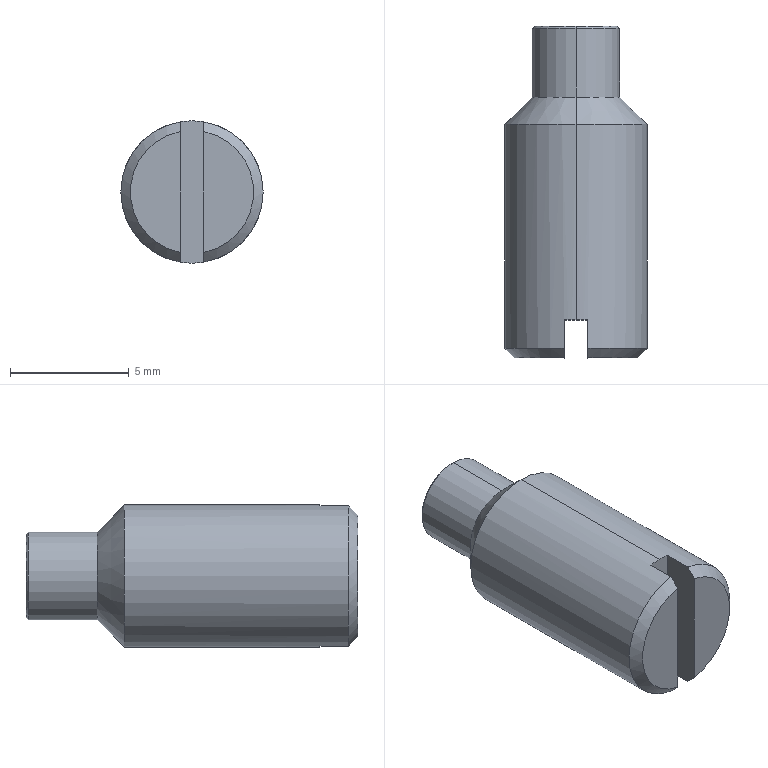Component | NX | GB_T_75_1985_SLOTTEDSETSCREW_M6X14 | 1 solid | 16 faces | box 6 x 14 x 6 mm | volume 321 mm3 | cone 6 | plane 6 | cylinder 4 | commonest cylinder face diameters 3.7 x2 6 x2
STEP:
#1=CARTESIAN_POINT('',(0.,0.,0.));
#2=DIRECTION('',(0.,0.,1.));
#3=DIRECTION('',(1.,0.,0.));
#4=AXIS2_PLACEMENT_3D('',#1,#2,#3);
#5=CARTESIAN_POINT('',(4.835,-12.785,234.25));
#6=VERTEX_POINT('',#5);
#7=CARTESIAN_POINT('',(4.835,-12.785,237.75));
#8=VERTEX_POINT('',#7);
#9=CARTESIAN_POINT('',(4.835,-12.785,236.));
#10=DIRECTION('',(0.,1.,0.));
#11=DIRECTION('',(0.,0.,1.));
#12=AXIS2_PLACEMENT_3D('',#9,#10,#11);
#13=CIRCLE('',#12,1.75);
#14=CARTESIAN_POINT('',(4.835,-12.885,236.));
#15=DIRECTION('',(0.,-1.,0.));
#16=DIRECTION('',(0.,0.,-1.));
#17=AXIS2_PLACEMENT_3D('',#14,#15,#16);
#18=CONICAL_SURFACE('',#17,1.85,0.7854);
#19=CARTESIAN_POINT('',(9.425,-0.1));
#20=DIRECTION('',(-1.,0.));
#21=VECTOR('',#20,1.);
#22=LINE('',#19,#21);
#23=(GEOMETRIC_REPRESENTATION_CONTEXT(2)PARAMETRIC_REPRESENTATION_CONTEXT()REPRESENTATION_CONTEXT('',''));
#24=DEFINITIONAL_REPRESENTATION('',(#22),#23);
#25=PCURVE('',#18,#24);
#26=CARTESIAN_POINT('',(2.985,-12.785,236.));
#27=DIRECTION('',(0.,-1.,0.));
#28=DIRECTION('',(0.,0.,-1.));
#29=AXIS2_PLACEMENT_3D('',#26,#27,#28);
#30=PLANE('',#29);
#31=CARTESIAN_POINT('',(-1.75,1.85));
#32=CARTESIAN_POINT('',(-1.75,4.881));
#33=CARTESIAN_POINT('',(0.875,3.366));
#34=CARTESIAN_POINT('',(3.5,1.85));
#35=CARTESIAN_POINT('',(0.875,0.3345));
#36=CARTESIAN_POINT('',(-1.75,-1.181));
#37=CARTESIAN_POINT('',(-1.75,1.85));
#38=(BOUNDED_CURVE()B_SPLINE_CURVE(2,(#31,#32,#33,#34,#35,#36,#37),.UNSPECIFIED.,.T.,.F.)B_SPLINE_CURVE_WITH_KNOTS((1,2,2,2,2,1),(-2.094,0.,2.094,4.189,6.283,8.378),.UNSPECIFIED.)CURVE()GEOMETRIC_REPRESENTATION_ITEM()RATIONAL_B_SPLINE_CURVE((1.,0.5,1.,0.5,1.,0.5,1.))REPRESENTATION_ITEM(''));
#39=(GEOMETRIC_REPRESENTATION_CONTEXT(2)PARAMETRIC_REPRESENTATION_CONTEXT()REPRESENTATION_CONTEXT('',''));
#40=DEFINITIONAL_REPRESENTATION('',(#38),#39);
#41=PCURVE('',#30,#40);
#42=SURFACE_CURVE('',#13,(#25,#41),.PCURVE_S1.);
#43=EDGE_CURVE('',#6,#8,#42,.T.);
#44=ORIENTED_EDGE('',*,*,#43,.F.);
#45=CARTESIAN_POINT('',(4.835,-12.885,234.15));
#46=VERTEX_POINT('',#45);
#47=CARTESIAN_POINT('',(4.835,-12.885,234.15));
#48=DIRECTION('',(-0.,-0.7071,-0.7071));
#49=VECTOR('',#48,1.);
#50=LINE('',#47,#49);
#51=CARTESIAN_POINT('',(6.283,-0.));
#52=DIRECTION('',(0.,1.));
#53=VECTOR('',#52,1.);
#54=LINE('',#51,#53);
#55=(GEOMETRIC_REPRESENTATION_CONTEXT(2)PARAMETRIC_REPRESENTATION_CONTEXT()REPRESENTATION_CONTEXT('',''));
#56=DEFINITIONAL_REPRESENTATION('',(#54),#55);
#57=PCURVE('',#18,#56);
#58=CARTESIAN_POINT('',(4.835,-12.885,236.));
#59=DIRECTION('',(0.,-1.,0.));
#60=DIRECTION('',(0.,0.,-1.));
#61=AXIS2_PLACEMENT_3D('',#58,#59,#60);
#62=CONICAL_SURFACE('',#61,1.85,0.7854);
#63=CARTESIAN_POINT('',(0.,-0.));
#64=DIRECTION('',(0.,1.));
#65=VECTOR('',#64,1.);
#66=LINE('',#63,#65);
#67=(GEOMETRIC_REPRESENTATION_CONTEXT(2)PARAMETRIC_REPRESENTATION_CONTEXT()REPRESENTATION_CONTEXT('',''));
#68=DEFINITIONAL_REPRESENTATION('',(#66),#67);
#69=PCURVE('',#62,#68);
#70=SURFACE_CURVE('',#50,(#57,#69),.PCURVE_S1.);
#71=EDGE_CURVE('',#6,#46,#70,.T.);
#72=ORIENTED_EDGE('',*,*,#71,.T.);
#73=CARTESIAN_POINT('',(4.835,-12.885,237.85));
#74=VERTEX_POINT('',#73);
#75=CARTESIAN_POINT('',(4.835,-12.885,236.));
#76=DIRECTION('',(0.,-1.,0.));
#77=DIRECTION('',(0.,0.,1.));
#78=AXIS2_PLACEMENT_3D('',#75,#76,#77);
#79=CIRCLE('',#78,1.85);
#80=CARTESIAN_POINT('',(3.142,-0.));
#81=DIRECTION('',(1.,0.));
#82=VECTOR('',#81,1.);
#83=LINE('',#80,#82);
#84=(GEOMETRIC_REPRESENTATION_CONTEXT(2)PARAMETRIC_REPRESENTATION_CONTEXT()REPRESENTATION_CONTEXT('',''));
#85=DEFINITIONAL_REPRESENTATION('',(#83),#84);
#86=PCURVE('',#18,#85);
#87=CARTESIAN_POINT('',(4.835,-28.21,236.));
#88=DIRECTION('',(0.,-1.,0.));
#89=DIRECTION('',(0.,0.,-1.));
#90=AXIS2_PLACEMENT_3D('',#87,#88,#89);
#91=CYLINDRICAL_SURFACE('',#90,1.85);
#92=CARTESIAN_POINT('',(3.142,-15.325));
#93=DIRECTION('',(1.,0.));
#94=VECTOR('',#93,1.);
#95=LINE('',#92,#94);
#96=(GEOMETRIC_REPRESENTATION_CONTEXT(2)PARAMETRIC_REPRESENTATION_CONTEXT()REPRESENTATION_CONTEXT('',''));
#97=DEFINITIONAL_REPRESENTATION('',(#95),#96);
#98=PCURVE('',#91,#97);
#99=SURFACE_CURVE('',#79,(#86,#98),.PCURVE_S1.);
#100=EDGE_CURVE('',#74,#46,#99,.T.);
#101=ORIENTED_EDGE('',*,*,#100,.F.);
#102=CARTESIAN_POINT('',(4.835,-12.885,237.85));
#103=DIRECTION('',(0.,-0.7071,0.7071));
#104=VECTOR('',#103,1.);
#105=LINE('',#102,#104);
#106=CARTESIAN_POINT('',(3.142,-0.));
#107=DIRECTION('',(0.,1.));
#108=VECTOR('',#107,1.);
#109=LINE('',#106,#108);
#110=(GEOMETRIC_REPRESENTATION_CONTEXT(2)PARAMETRIC_REPRESENTATION_CONTEXT()REPRESENTATION_CONTEXT('',''));
#111=DEFINITIONAL_REPRESENTATION('',(#109),#110);
#112=PCURVE('',#18,#111);
#113=CARTESIAN_POINT('',(3.142,-0.));
#114=DIRECTION('',(0.,1.));
#115=VECTOR('',#114,1.);
#116=LINE('',#113,#115);
#117=(GEOMETRIC_REPRESENTATION_CONTEXT(2)PARAMETRIC_REPRESENTATION_CONTEXT()REPRESENTATION_CONTEXT('',''));
#118=DEFINITIONAL_REPRESENTATION('',(#116),#117);
#119=PCURVE('',#62,#118);
#120=SURFACE_CURVE('',#105,(#112,#119),.PCURVE_S1.);
#121=EDGE_CURVE('',#8,#74,#120,.T.);
#122=ORIENTED_EDGE('',*,*,#121,.F.);
#123=EDGE_LOOP('',(#44,#72,#101,#122));
#124=FACE_BOUND('',#123,.T.);
#125=ADVANCED_FACE('',(#124),#18,.T.);
#126=ORIENTED_EDGE('',*,*,#100,.T.);
#127=CARTESIAN_POINT('',(4.835,-15.785,234.15));
#128=VERTEX_POINT('',#127);
#129=CARTESIAN_POINT('',(4.835,-28.21,234.15));
#130=DIRECTION('',(0.,-1.,0.));
#131=VECTOR('',#130,1.);
#132=LINE('',#129,#131);
#133=CARTESIAN_POINT('',(6.283,0.));
#134=DIRECTION('',(0.,1.));
#135=VECTOR('',#134,1.);
#136=LINE('',#133,#135);
#137=(GEOMETRIC_REPRESENTATION_CONTEXT(2)PARAMETRIC_REPRESENTATION_CONTEXT()REPRESENTATION_CONTEXT('',''));
#138=DEFINITIONAL_REPRESENTATION('',(#136),#137);
#139=PCURVE('',#91,#138);
#140=CARTESIAN_POINT('',(4.835,-28.21,236.));
#141=DIRECTION('',(0.,-1.,0.));
#142=DIRECTION('',(0.,0.,-1.));
#143=AXIS2_PLACEMENT_3D('',#140,#141,#142);
#144=CYLINDRICAL_SURFACE('',#143,1.85);
#145=CARTESIAN_POINT('',(0.,0.));
#146=DIRECTION('',(0.,1.));
#147=VECTOR('',#146,1.);
#148=LINE('',#145,#147);
#149=(GEOMETRIC_REPRESENTATION_CONTEXT(2)PARAMETRIC_REPRESENTATION_CONTEXT()REPRESENTATION_CONTEXT('',''));
#150=DEFINITIONAL_REPRESENTATION('',(#148),#149);
#151=PCURVE('',#144,#150);
#152=SURFACE_CURVE('',#132,(#139,#151),.PCURVE_S1.);
#153=EDGE_CURVE('',#46,#128,#152,.T.);
#154=ORIENTED_EDGE('',*,*,#153,.T.);
#155=CARTESIAN_POINT('',(4.835,-15.785,237.85));
#156=VERTEX_POINT('',#155);
#157=CARTESIAN_POINT('',(4.835,-15.785,236.));
#158=DIRECTION('',(0.,-1.,0.));
#159=DIRECTION('',(0.,0.,1.));
#160=AXIS2_PLACEMENT_3D('',#157,#158,#159);
#161=CIRCLE('',#160,1.85);
#162=CARTESIAN_POINT('',(3.142,-12.425));
#163=DIRECTION('',(1.,0.));
#164=VECTOR('',#163,1.);
#165=LINE('',#162,#164);
#166=(GEOMETRIC_REPRESENTATION_CONTEXT(2)PARAMETRIC_REPRESENTATION_CONTEXT()REPRESENTATION_CONTEXT('',''));
#167=DEFINITIONAL_REPRESENTATION('',(#165),#166);
#168=PCURVE('',#91,#167);
#169=CARTESIAN_POINT('',(4.835,-15.785,236.));
#170=DIRECTION('',(0.,-1.,0.));
#171=DIRECTION('',(0.,0.,-1.));
#172=AXIS2_PLACEMENT_3D('',#169,#170,#171);
#173=CONICAL_SURFACE('',#172,1.85,0.7854);
#174=CARTESIAN_POINT('',(3.142,-0.));
#175=DIRECTION('',(1.,0.));
#176=VECTOR('',#175,1.);
#177=LINE('',#174,#176);
#178=(GEOMETRIC_REPRESENTATION_CONTEXT(2)PARAMETRIC_REPRESENTATION_CONTEXT()REPRESENTATION_CONTEXT('',''));
#179=DEFINITIONAL_REPRESENTATION('',(#177),#178);
#180=PCURVE('',#173,#179);
#181=SURFACE_CURVE('',#161,(#168,#180),.PCURVE_S1.);
#182=EDGE_CURVE('',#156,#128,#181,.T.);
#183=ORIENTED_EDGE('',*,*,#182,.F.);
#184=CARTESIAN_POINT('',(4.835,-28.21,237.85));
#185=DIRECTION('',(0.,-1.,0.));
#186=VECTOR('',#185,1.);
#187=LINE('',#184,#186);
#188=CARTESIAN_POINT('',(3.142,0.));
#189=DIRECTION('',(0.,1.));
#190=VECTOR('',#189,1.);
#191=LINE('',#188,#190);
#192=(GEOMETRIC_REPRESENTATION_CONTEXT(2)PARAMETRIC_REPRESENTATION_CONTEXT()REPRESENTATION_CONTEXT('',''));
#193=DEFINITIONAL_REPRESENTATION('',(#191),#192);
#194=PCURVE('',#91,#193);
#195=CARTESIAN_POINT('',(3.142,0.));
#196=DIRECTION('',(0.,1.));
#197=VECTOR('',#196,1.);
#198=LINE('',#195,#197);
#199=(GEOMETRIC_REPRESENTATION_CONTEXT(2)PARAMETRIC_REPRESENTATION_CONTEXT()REPRESENTATION_CONTEXT('',''));
#200=DEFINITIONAL_REPRESENTATION('',(#198),#199);
#201=PCURVE('',#144,#200);
#202=SURFACE_CURVE('',#187,(#194,#201),.PCURVE_S1.);
#203=EDGE_CURVE('',#74,#156,#202,.T.);
#204=ORIENTED_EDGE('',*,*,#203,.F.);
#205=EDGE_LOOP('',(#126,#154,#183,#204));
#206=FACE_BOUND('',#205,.T.);
#207=ADVANCED_FACE('',(#206),#91,.T.);
#208=ORIENTED_EDGE('',*,*,#182,.T.);
#209=CARTESIAN_POINT('',(4.835,-16.935,233.));
#210=VERTEX_POINT('',#209);
#211=CARTESIAN_POINT('',(4.835,-15.785,234.15));
#212=DIRECTION('',(-0.,-0.7071,-0.7071));
#213=VECTOR('',#212,1.);
#214=LINE('',#211,#213);
#215=CARTESIAN_POINT('',(6.283,-0.));
#216=DIRECTION('',(0.,1.));
#217=VECTOR('',#216,1.);
#218=LINE('',#215,#217);
#219=(GEOMETRIC_REPRESENTATION_CONTEXT(2)PARAMETRIC_REPRESENTATION_CONTEXT()REPRESENTATION_CONTEXT('',''));
#220=DEFINITIONAL_REPRESENTATION('',(#218),#219);
#221=PCURVE('',#173,#220);
#222=CARTESIAN_POINT('',(4.835,-15.785,236.));
#223=DIRECTION('',(0.,-1.,0.));
#224=DIRECTION('',(0.,0.,-1.));
#225=AXIS2_PLACEMENT_3D('',#222,#223,#224);
#226=CONICAL_SURFACE('',#225,1.85,0.7854);
#227=CARTESIAN_POINT('',(0.,-0.));
#228=DIRECTION('',(0.,1.));
#229=VECTOR('',#228,1.);
#230=LINE('',#227,#229);
#231=(GEOMETRIC_REPRESENTATION_CONTEXT(2)PARAMETRIC_REPRESENTATION_CONTEXT()REPRESENTATION_CONTEXT('',''));
#232=DEFINITIONAL_REPRESENTATION('',(#230),#231);
#233=PCURVE('',#226,#232);
#234=SURFACE_CURVE('',#214,(#221,#233),.PCURVE_S1.);
#235=EDGE_CURVE('',#128,#210,#234,.T.);
#236=ORIENTED_EDGE('',*,*,#235,.T.);
#237=CARTESIAN_POINT('',(4.835,-16.935,239.));
#238=VERTEX_POINT('',#237);
#239=CARTESIAN_POINT('',(4.835,-16.935,236.));
#240=DIRECTION('',(0.,-1.,0.));
#241=DIRECTION('',(0.,0.,1.));
#242=AXIS2_PLACEMENT_3D('',#239,#240,#241);
#243=CIRCLE('',#242,3.);
#244=CARTESIAN_POINT('',(3.142,1.15));
#245=DIRECTION('',(1.,0.));
#246=VECTOR('',#245,1.);
#247=LINE('',#244,#246);
#248=(GEOMETRIC_REPRESENTATION_CONTEXT(2)PARAMETRIC_REPRESENTATION_CONTEXT()REPRESENTATION_CONTEXT('',''));
#249=DEFINITIONAL_REPRESENTATION('',(#247),#248);
#250=PCURVE('',#173,#249);
#251=CARTESIAN_POINT('',(4.835,-28.21,236.));
#252=DIRECTION('',(0.,-1.,0.));
#253=DIRECTION('',(0.,0.,-1.));
#254=AXIS2_PLACEMENT_3D('',#251,#252,#253);
#255=CYLINDRICAL_SURFACE('',#254,3.);
#256=CARTESIAN_POINT('',(3.142,-11.275));
#257=DIRECTION('',(1.,0.));
#258=VECTOR('',#257,1.);
#259=LINE('',#256,#258);
#260=(GEOMETRIC_REPRESENTATION_CONTEXT(2)PARAMETRIC_REPRESENTATION_CONTEXT()REPRESENTATION_CONTEXT('',''));
#261=DEFINITIONAL_REPRESENTATION('',(#259),#260);
#262=PCURVE('',#255,#261);
#263=SURFACE_CURVE('',#243,(#250,#262),.PCURVE_S1.);
#264=EDGE_CURVE('',#238,#210,#263,.T.);
#265=ORIENTED_EDGE('',*,*,#264,.F.);
#266=CARTESIAN_POINT('',(4.835,-15.785,237.85));
#267=DIRECTION('',(0.,-0.7071,0.7071));
#268=VECTOR('',#267,1.);
#269=LINE('',#266,#268);
#270=CARTESIAN_POINT('',(3.142,-0.));
#271=DIRECTION('',(0.,1.));
#272=VECTOR('',#271,1.);
#273=LINE('',#270,#272);
#274=(GEOMETRIC_REPRESENTATION_CONTEXT(2)PARAMETRIC_REPRESENTATION_CONTEXT()REPRESENTATION_CONTEXT('',''));
#275=DEFINITIONAL_REPRESENTATION('',(#273),#274);
#276=PCURVE('',#173,#275);
#277=CARTESIAN_POINT('',(3.142,-0.));
#278=DIRECTION('',(0.,1.));
#279=VECTOR('',#278,1.);
#280=LINE('',#277,#279);
#281=(GEOMETRIC_REPRESENTATION_CONTEXT(2)PARAMETRIC_REPRESENTATION_CONTEXT()REPRESENTATION_CONTEXT('',''));
#282=DEFINITIONAL_REPRESENTATION('',(#280),#281);
#283=PCURVE('',#226,#282);
#284=SURFACE_CURVE('',#269,(#276,#283),.PCURVE_S1.);
#285=EDGE_CURVE('',#156,#238,#284,.T.);
#286=ORIENTED_EDGE('',*,*,#285,.F.);
#287=EDGE_LOOP('',(#208,#236,#265,#286));
#288=FACE_BOUND('',#287,.T.);
#289=ADVANCED_FACE('',(#288),#173,.T.);
#290=ORIENTED_EDGE('',*,*,#264,.T.);
#291=CARTESIAN_POINT('',(4.835,-25.185,233.));
#292=VERTEX_POINT('',#291);
#293=CARTESIAN_POINT('',(4.835,-28.21,233.));
#294=DIRECTION('',(0.,-1.,0.));
#295=VECTOR('',#294,1.);
#296=LINE('',#293,#295);
#297=CARTESIAN_POINT('',(6.283,0.));
#298=DIRECTION('',(0.,1.));
#299=VECTOR('',#298,1.);
#300=LINE('',#297,#299);
#301=(GEOMETRIC_REPRESENTATION_CONTEXT(2)PARAMETRIC_REPRESENTATION_CONTEXT()REPRESENTATION_CONTEXT('',''));
#302=DEFINITIONAL_REPRESENTATION('',(#300),#301);
#303=PCURVE('',#255,#302);
#304=CARTESIAN_POINT('',(4.835,-28.21,236.));
#305=DIRECTION('',(0.,-1.,0.));
#306=DIRECTION('',(0.,0.,-1.));
#307=AXIS2_PLACEMENT_3D('',#304,#305,#306);
#308=CYLINDRICAL_SURFACE('',#307,3.);
#309=CARTESIAN_POINT('',(0.,0.));
#310=DIRECTION('',(0.,1.));
#311=VECTOR('',#310,1.);
#312=LINE('',#309,#311);
#313=(GEOMETRIC_REPRESENTATION_CONTEXT(2)PARAMETRIC_REPRESENTATION_CONTEXT()REPRESENTATION_CONTEXT('',''));
#314=DEFINITIONAL_REPRESENTATION('',(#312),#313);
#315=PCURVE('',#308,#314);
#316=SURFACE_CURVE('',#296,(#303,#315),.PCURVE_S1.);
#317=EDGE_CURVE('',#210,#292,#316,.T.);
#318=ORIENTED_EDGE('',*,*,#317,.T.);
#319=CARTESIAN_POINT('',(4.335,-25.185,233.042));
#320=VERTEX_POINT('',#319);
#321=CARTESIAN_POINT('',(4.835,-25.185,236.));
#322=DIRECTION('',(0.,1.,0.));
#323=DIRECTION('',(0.,0.,-1.));
#324=AXIS2_PLACEMENT_3D('',#321,#322,#323);
#325=CIRCLE('',#324,3.);
#326=CARTESIAN_POINT('',(6.283,-3.025));
#327=DIRECTION('',(-1.,0.));
#328=VECTOR('',#327,1.);
#329=LINE('',#326,#328);
#330=(GEOMETRIC_REPRESENTATION_CONTEXT(2)PARAMETRIC_REPRESENTATION_CONTEXT()REPRESENTATION_CONTEXT('',''));
#331=DEFINITIONAL_REPRESENTATION('',(#329),#330);
#332=PCURVE('',#255,#331);
#333=CARTESIAN_POINT('',(4.335,-25.185,186.));
#334=DIRECTION('',(0.,1.,0.));
#335=DIRECTION('',(0.,0.,1.));
#336=AXIS2_PLACEMENT_3D('',#333,#334,#335);
#337=PLANE('',#336);
#338=CARTESIAN_POINT('',(50.,0.5));
#339=DIRECTION('',(-1.,0.));
#340=AXIS2_PLACEMENT_2D('',#338,#339);
#341=CIRCLE('',#340,3.);
#342=(GEOMETRIC_REPRESENTATION_CONTEXT(2)PARAMETRIC_REPRESENTATION_CONTEXT()REPRESENTATION_CONTEXT('',''));
#343=DEFINITIONAL_REPRESENTATION('',(#341),#342);
#344=PCURVE('',#337,#343);
#345=SURFACE_CURVE('',#325,(#332,#344),.PCURVE_S1.);
#346=EDGE_CURVE('',#292,#320,#345,.T.);
#347=ORIENTED_EDGE('',*,*,#346,.T.);
#348=CARTESIAN_POINT('',(4.335,-26.383,233.042));
#349=VERTEX_POINT('',#348);
#350=CARTESIAN_POINT('',(4.335,-28.21,233.042));
#351=DIRECTION('',(0.,-1.,0.));
#352=VECTOR('',#351,1.);
#353=LINE('',#350,#352);
#354=CARTESIAN_POINT('',(6.116,0.));
#355=DIRECTION('',(0.,1.));
#356=VECTOR('',#355,1.);
#357=LINE('',#354,#356);
#358=(GEOMETRIC_REPRESENTATION_CONTEXT(2)PARAMETRIC_REPRESENTATION_CONTEXT()REPRESENTATION_CONTEXT('',''));
#359=DEFINITIONAL_REPRESENTATION('',(#357),#358);
#360=PCURVE('',#255,#359);
#361=CARTESIAN_POINT('',(4.335,-26.785,186.));
#362=DIRECTION('',(-1.,0.,0.));
#363=DIRECTION('',(0.,0.,-1.));
#364=AXIS2_PLACEMENT_3D('',#361,#362,#363);
#365=PLANE('',#364);
#366=CARTESIAN_POINT('',(-47.042,1.425));
#367=DIRECTION('',(0.,1.));
#368=VECTOR('',#367,1.);
#369=LINE('',#366,#368);
#370=(GEOMETRIC_REPRESENTATION_CONTEXT(2)PARAMETRIC_REPRESENTATION_CONTEXT()REPRESENTATION_CONTEXT('',''));
#371=DEFINITIONAL_REPRESENTATION('',(#369),#370);
#372=PCURVE('',#365,#371);
#373=SURFACE_CURVE('',#353,(#360,#372),.PCURVE_S1.);
#374=EDGE_CURVE('',#320,#349,#373,.T.);
#375=ORIENTED_EDGE('',*,*,#374,.T.);
#376=CARTESIAN_POINT('',(4.335,-26.383,238.958));
#377=VERTEX_POINT('',#376);
#378=CARTESIAN_POINT('',(4.835,-26.383,236.));
#379=DIRECTION('',(0.,-1.,0.));
#380=DIRECTION('',(0.,0.,1.));
#381=AXIS2_PLACEMENT_3D('',#378,#379,#380);
#382=CIRCLE('',#381,3.);
#383=CARTESIAN_POINT('',(3.142,-1.827));
#384=DIRECTION('',(1.,0.));
#385=VECTOR('',#384,1.);
#386=LINE('',#383,#385);
#387=(GEOMETRIC_REPRESENTATION_CONTEXT(2)PARAMETRIC_REPRESENTATION_CONTEXT()REPRESENTATION_CONTEXT('',''));
#388=DEFINITIONAL_REPRESENTATION('',(#386),#387);
#389=PCURVE('',#255,#388);
#390=CARTESIAN_POINT('',(4.835,-26.383,236.));
#391=DIRECTION('',(0.,1.,0.));
#392=DIRECTION('',(0.,0.,1.));
#393=AXIS2_PLACEMENT_3D('',#390,#391,#392);
#394=CONICAL_SURFACE('',#393,3.,0.7854);
#395=CARTESIAN_POINT('',(6.283,0.));
#396=DIRECTION('',(-1.,0.));
#397=VECTOR('',#396,1.);
#398=LINE('',#395,#397);
#399=(GEOMETRIC_REPRESENTATION_CONTEXT(2)PARAMETRIC_REPRESENTATION_CONTEXT()REPRESENTATION_CONTEXT('',''));
#400=DEFINITIONAL_REPRESENTATION('',(#398),#399);
#401=PCURVE('',#394,#400);
#402=SURFACE_CURVE('',#382,(#389,#401),.PCURVE_S1.);
#403=EDGE_CURVE('',#377,#349,#402,.T.);
#404=ORIENTED_EDGE('',*,*,#403,.F.);
#405=CARTESIAN_POINT('',(4.335,-25.185,238.958));
#406=VERTEX_POINT('',#405);
#407=CARTESIAN_POINT('',(4.335,-28.21,238.958));
#408=DIRECTION('',(0.,1.,0.));
#409=VECTOR('',#408,1.);
#410=LINE('',#407,#409);
#411=CARTESIAN_POINT('',(3.309,0.));
#412=DIRECTION('',(0.,-1.));
#413=VECTOR('',#412,1.);
#414=LINE('',#411,#413);
#415=(GEOMETRIC_REPRESENTATION_CONTEXT(2)PARAMETRIC_REPRESENTATION_CONTEXT()REPRESENTATION_CONTEXT('',''));
#416=DEFINITIONAL_REPRESENTATION('',(#414),#415);
#417=PCURVE('',#255,#416);
#418=CARTESIAN_POINT('',(-52.958,1.425));
#419=DIRECTION('',(0.,-1.));
#420=VECTOR('',#419,1.);
#421=LINE('',#418,#420);
#422=(GEOMETRIC_REPRESENTATION_CONTEXT(2)PARAMETRIC_REPRESENTATION_CONTEXT()REPRESENTATION_CONTEXT('',''));
#423=DEFINITIONAL_REPRESENTATION('',(#421),#422);
#424=PCURVE('',#365,#423);
#425=SURFACE_CURVE('',#410,(#417,#424),.PCURVE_S1.);
#426=EDGE_CURVE('',#377,#406,#425,.T.);
#427=ORIENTED_EDGE('',*,*,#426,.T.);
#428=CARTESIAN_POINT('',(4.835,-25.185,239.));
#429=VERTEX_POINT('',#428);
#430=CARTESIAN_POINT('',(4.835,-25.185,236.));
#431=DIRECTION('',(0.,1.,0.));
#432=DIRECTION('',(0.,0.,-1.));
#433=AXIS2_PLACEMENT_3D('',#430,#431,#432);
#434=CIRCLE('',#433,3.);
#435=CARTESIAN_POINT('',(6.283,-3.025));
#436=DIRECTION('',(-1.,0.));
#437=VECTOR('',#436,1.);
#438=LINE('',#435,#437);
#439=(GEOMETRIC_REPRESENTATION_CONTEXT(2)PARAMETRIC_REPRESENTATION_CONTEXT()REPRESENTATION_CONTEXT('',''));
#440=DEFINITIONAL_REPRESENTATION('',(#438),#439);
#441=PCURVE('',#255,#440);
#442=CARTESIAN_POINT('',(50.,0.5));
#443=DIRECTION('',(-1.,0.));
#444=AXIS2_PLACEMENT_2D('',#442,#443);
#445=CIRCLE('',#444,3.);
#446=(GEOMETRIC_REPRESENTATION_CONTEXT(2)PARAMETRIC_REPRESENTATION_CONTEXT()REPRESENTATION_CONTEXT('',''));
#447=DEFINITIONAL_REPRESENTATION('',(#445),#446);
#448=PCURVE('',#337,#447);
#449=SURFACE_CURVE('',#434,(#441,#448),.PCURVE_S1.);
#450=EDGE_CURVE('',#406,#429,#449,.T.);
#451=ORIENTED_EDGE('',*,*,#450,.T.);
#452=CARTESIAN_POINT('',(4.835,-28.21,239.));
#453=DIRECTION('',(0.,-1.,0.));
#454=VECTOR('',#453,1.);
#455=LINE('',#452,#454);
#456=CARTESIAN_POINT('',(3.142,0.));
#457=DIRECTION('',(0.,1.));
#458=VECTOR('',#457,1.);
#459=LINE('',#456,#458);
#460=(GEOMETRIC_REPRESENTATION_CONTEXT(2)PARAMETRIC_REPRESENTATION_CONTEXT()REPRESENTATION_CONTEXT('',''));
#461=DEFINITIONAL_REPRESENTATION('',(#459),#460);
#462=PCURVE('',#255,#461);
#463=CARTESIAN_POINT('',(3.142,0.));
#464=DIRECTION('',(0.,1.));
#465=VECTOR('',#464,1.);
#466=LINE('',#463,#465);
#467=(GEOMETRIC_REPRESENTATION_CONTEXT(2)PARAMETRIC_REPRESENTATION_CONTEXT()REPRESENTATION_CONTEXT('',''));
#468=DEFINITIONAL_REPRESENTATION('',(#466),#467);
#469=PCURVE('',#308,#468);
#470=SURFACE_CURVE('',#455,(#462,#469),.PCURVE_S1.);
#471=EDGE_CURVE('',#238,#429,#470,.T.);
#472=ORIENTED_EDGE('',*,*,#471,.F.);
#473=EDGE_LOOP('',(#290,#318,#347,#375,#404,#427,#451,#472));
#474=FACE_BOUND('',#473,.T.);
#475=ADVANCED_FACE('',(#474),#255,.T.);
#476=CARTESIAN_POINT('',(4.335,-26.785,238.549));
#477=VERTEX_POINT('',#476);
#478=CARTESIAN_POINT('',(4.335,-26.785,233.451));
#479=VERTEX_POINT('',#478);
#480=CARTESIAN_POINT('',(4.835,-26.785,236.));
#481=DIRECTION('',(0.,-1.,0.));
#482=DIRECTION('',(0.,0.,1.));
#483=AXIS2_PLACEMENT_3D('',#480,#481,#482);
#484=CIRCLE('',#483,2.598);
#485=CARTESIAN_POINT('',(4.835,-26.785,236.));
#486=DIRECTION('',(0.,1.,0.));
#487=DIRECTION('',(0.,0.,1.));
#488=AXIS2_PLACEMENT_3D('',#485,#486,#487);
#489=PLANE('',#488);
#490=CARTESIAN_POINT('',(2.598,0.));
#491=CARTESIAN_POINT('',(2.598,-4.5));
#492=CARTESIAN_POINT('',(-1.299,-2.25));
#493=CARTESIAN_POINT('',(-5.196,-0.));
#494=CARTESIAN_POINT('',(-1.299,2.25));
#495=CARTESIAN_POINT('',(2.598,4.5));
#496=CARTESIAN_POINT('',(2.598,0.));
#497=(BOUNDED_CURVE()B_SPLINE_CURVE(2,(#490,#491,#492,#493,#494,#495,#496),.UNSPECIFIED.,.T.,.F.)B_SPLINE_CURVE_WITH_KNOTS((1,2,2,2,2,1),(-2.094,0.,2.094,4.189,6.283,8.378),.UNSPECIFIED.)CURVE()GEOMETRIC_REPRESENTATION_ITEM()RATIONAL_B_SPLINE_CURVE((1.,0.5,1.,0.5,1.,0.5,1.))REPRESENTATION_ITEM(''));
#498=(GEOMETRIC_REPRESENTATION_CONTEXT(2)PARAMETRIC_REPRESENTATION_CONTEXT()REPRESENTATION_CONTEXT('',''));
#499=DEFINITIONAL_REPRESENTATION('',(#497),#498);
#500=PCURVE('',#489,#499);
#501=CARTESIAN_POINT('',(6.283,-0.402));
#502=DIRECTION('',(-1.,0.));
#503=VECTOR('',#502,1.);
#504=LINE('',#501,#503);
#505=(GEOMETRIC_REPRESENTATION_CONTEXT(2)PARAMETRIC_REPRESENTATION_CONTEXT()REPRESENTATION_CONTEXT('',''));
#506=DEFINITIONAL_REPRESENTATION('',(#504),#505);
#507=PCURVE('',#394,#506);
#508=SURFACE_CURVE('',#484,(#500,#507),.PCURVE_S1.);
#509=EDGE_CURVE('',#477,#479,#508,.T.);
#510=ORIENTED_EDGE('',*,*,#509,.T.);
#511=CARTESIAN_POINT('',(4.335,-26.785,186.));
#512=DIRECTION('',(0.,0.,1.));
#513=VECTOR('',#512,1.);
#514=LINE('',#511,#513);
#515=CARTESIAN_POINT('',(-50.,-0.5));
#516=DIRECTION('',(1.,0.));
#517=VECTOR('',#516,1.);
#518=LINE('',#515,#517);
#519=(GEOMETRIC_REPRESENTATION_CONTEXT(2)PARAMETRIC_REPRESENTATION_CONTEXT()REPRESENTATION_CONTEXT('',''));
#520=DEFINITIONAL_REPRESENTATION('',(#518),#519);
#521=PCURVE('',#489,#520);
#522=CARTESIAN_POINT('',(0.,0.));
#523=DIRECTION('',(-1.,0.));
#524=VECTOR('',#523,1.);
#525=LINE('',#522,#524);
#526=(GEOMETRIC_REPRESENTATION_CONTEXT(2)PARAMETRIC_REPRESENTATION_CONTEXT()REPRESENTATION_CONTEXT('',''));
#527=DEFINITIONAL_REPRESENTATION('',(#525),#526);
#528=PCURVE('',#365,#527);
#529=SURFACE_CURVE('',#514,(#521,#528),.PCURVE_S1.);
#530=EDGE_CURVE('',#479,#477,#529,.T.);
#531=ORIENTED_EDGE('',*,*,#530,.T.);
#532=EDGE_LOOP('',(#510,#531));
#533=FACE_BOUND('',#532,.T.);
#534=ADVANCED_FACE('',(#533),#489,.F.);
#535=ORIENTED_EDGE('',*,*,#403,.T.);
#536=CARTESIAN_POINT('',(4.335,-26.383,233.042));
#537=CARTESIAN_POINT('',(4.335,-26.517,233.178));
#538=CARTESIAN_POINT('',(4.335,-26.651,233.314));
#539=CARTESIAN_POINT('',(4.335,-26.785,233.451));
#540=B_SPLINE_CURVE_WITH_KNOTS('',3,(#536,#537,#538,#539),.UNSPECIFIED.,.F.,.F.,(4,4),(0.,1.),.PIECEWISE_BEZIER_KNOTS.);
#541=CARTESIAN_POINT('',(3.309,0.));
#542=CARTESIAN_POINT('',(3.335,-0.402));
#543=B_SPLINE_CURVE_WITH_KNOTS('',1,(#541,#542),.UNSPECIFIED.,.F.,.F.,(2,2),(0.,1.),.PIECEWISE_BEZIER_KNOTS.);
#544=(GEOMETRIC_REPRESENTATION_CONTEXT(2)PARAMETRIC_REPRESENTATION_CONTEXT()REPRESENTATION_CONTEXT('',''));
#545=DEFINITIONAL_REPRESENTATION('',(#543),#544);
#546=PCURVE('',#394,#545);
#547=CARTESIAN_POINT('',(-47.042,-0.402));
#548=CARTESIAN_POINT('',(-47.178,-0.2678));
#549=CARTESIAN_POINT('',(-47.314,-0.1338));
#550=CARTESIAN_POINT('',(-47.451,0.));
#551=B_SPLINE_CURVE_WITH_KNOTS('',3,(#547,#548,#549,#550),.UNSPECIFIED.,.F.,.F.,(4,4),(0.,1.),.PIECEWISE_BEZIER_KNOTS.);
#552=(GEOMETRIC_REPRESENTATION_CONTEXT(2)PARAMETRIC_REPRESENTATION_CONTEXT()REPRESENTATION_CONTEXT('',''));
#553=DEFINITIONAL_REPRESENTATION('',(#551),#552);
#554=PCURVE('',#365,#553);
#555=SURFACE_CURVE('',#540,(#546,#554),.PCURVE_S1.);
#556=EDGE_CURVE('',#349,#479,#555,.T.);
#557=ORIENTED_EDGE('',*,*,#556,.T.);
#558=ORIENTED_EDGE('',*,*,#509,.F.);
#559=CARTESIAN_POINT('',(4.335,-26.785,238.549));
#560=CARTESIAN_POINT('',(4.335,-26.651,238.686));
#561=CARTESIAN_POINT('',(4.335,-26.517,238.822));
#562=CARTESIAN_POINT('',(4.335,-26.383,238.958));
#563=B_SPLINE_CURVE_WITH_KNOTS('',3,(#559,#560,#561,#562),.UNSPECIFIED.,.F.,.F.,(4,4),(0.,1.),.PIECEWISE_BEZIER_KNOTS.);
#564=CARTESIAN_POINT('',(6.09,-0.402));
#565=CARTESIAN_POINT('',(6.116,0.));
#566=B_SPLINE_CURVE_WITH_KNOTS('',1,(#564,#565),.UNSPECIFIED.,.F.,.F.,(2,2),(0.,1.),.PIECEWISE_BEZIER_KNOTS.);
#567=(GEOMETRIC_REPRESENTATION_CONTEXT(2)PARAMETRIC_REPRESENTATION_CONTEXT()REPRESENTATION_CONTEXT('',''));
#568=DEFINITIONAL_REPRESENTATION('',(#566),#567);
#569=PCURVE('',#394,#568);
#570=CARTESIAN_POINT('',(-52.549,0.));
#571=CARTESIAN_POINT('',(-52.686,-0.1338));
#572=CARTESIAN_POINT('',(-52.822,-0.2678));
#573=CARTESIAN_POINT('',(-52.958,-0.402));
#574=B_SPLINE_CURVE_WITH_KNOTS('',3,(#570,#571,#572,#573),.UNSPECIFIED.,.F.,.F.,(4,4),(0.,1.),.PIECEWISE_BEZIER_KNOTS.);
#575=(GEOMETRIC_REPRESENTATION_CONTEXT(2)PARAMETRIC_REPRESENTATION_CONTEXT()REPRESENTATION_CONTEXT('',''));
#576=DEFINITIONAL_REPRESENTATION('',(#574),#575);
#577=PCURVE('',#365,#576);
#578=SURFACE_CURVE('',#563,(#569,#577),.PCURVE_S1.);
#579=EDGE_CURVE('',#477,#377,#578,.T.);
#580=ORIENTED_EDGE('',*,*,#579,.T.);
#581=EDGE_LOOP('',(#535,#557,#558,#580));
#582=FACE_BOUND('',#581,.T.);
#583=ADVANCED_FACE('',(#582),#394,.T.);
#584=CARTESIAN_POINT('',(5.335,-26.785,233.451));
#585=VERTEX_POINT('',#584);
#586=CARTESIAN_POINT('',(5.335,-26.785,238.549));
#587=VERTEX_POINT('',#586);
#588=CARTESIAN_POINT('',(4.835,-26.785,236.));
#589=DIRECTION('',(0.,-1.,0.));
#590=DIRECTION('',(0.,0.,1.));
#591=AXIS2_PLACEMENT_3D('',#588,#589,#590);
#592=CIRCLE('',#591,2.598);
#593=CARTESIAN_POINT('',(4.835,-26.785,236.));
#594=DIRECTION('',(0.,1.,0.));
#595=DIRECTION('',(0.,0.,1.));
#596=AXIS2_PLACEMENT_3D('',#593,#594,#595);
#597=PLANE('',#596);
#598=CARTESIAN_POINT('',(2.598,0.));
#599=CARTESIAN_POINT('',(2.598,-4.5));
#600=CARTESIAN_POINT('',(-1.299,-2.25));
#601=CARTESIAN_POINT('',(-5.196,-0.));
#602=CARTESIAN_POINT('',(-1.299,2.25));
#603=CARTESIAN_POINT('',(2.598,4.5));
#604=CARTESIAN_POINT('',(2.598,0.));
#605=(BOUNDED_CURVE()B_SPLINE_CURVE(2,(#598,#599,#600,#601,#602,#603,#604),.UNSPECIFIED.,.T.,.F.)B_SPLINE_CURVE_WITH_KNOTS((1,2,2,2,2,1),(-2.094,0.,2.094,4.189,6.283,8.378),.UNSPECIFIED.)CURVE()GEOMETRIC_REPRESENTATION_ITEM()RATIONAL_B_SPLINE_CURVE((1.,0.5,1.,0.5,1.,0.5,1.))REPRESENTATION_ITEM(''));
#606=(GEOMETRIC_REPRESENTATION_CONTEXT(2)PARAMETRIC_REPRESENTATION_CONTEXT()REPRESENTATION_CONTEXT('',''));
#607=DEFINITIONAL_REPRESENTATION('',(#605),#606);
#608=PCURVE('',#597,#607);
#609=CARTESIAN_POINT('',(4.835,-26.383,236.));
#610=DIRECTION('',(0.,1.,0.));
#611=DIRECTION('',(0.,0.,1.));
#612=AXIS2_PLACEMENT_3D('',#609,#610,#611);
#613=CONICAL_SURFACE('',#612,3.,0.7854);
#614=CARTESIAN_POINT('',(6.283,-0.402));
#615=DIRECTION('',(-1.,0.));
#616=VECTOR('',#615,1.);
#617=LINE('',#614,#616);
#618=(GEOMETRIC_REPRESENTATION_CONTEXT(2)PARAMETRIC_REPRESENTATION_CONTEXT()REPRESENTATION_CONTEXT('',''));
#619=DEFINITIONAL_REPRESENTATION('',(#617),#618);
#620=PCURVE('',#613,#619);
#621=SURFACE_CURVE('',#592,(#608,#620),.PCURVE_S1.);
#622=EDGE_CURVE('',#585,#587,#621,.T.);
#623=ORIENTED_EDGE('',*,*,#622,.T.);
#624=CARTESIAN_POINT('',(5.335,-26.785,186.));
#625=DIRECTION('',(0.,0.,1.));
#626=VECTOR('',#625,1.);
#627=LINE('',#624,#626);
#628=CARTESIAN_POINT('',(-50.,0.5));
#629=DIRECTION('',(1.,0.));
#630=VECTOR('',#629,1.);
#631=LINE('',#628,#630);
#632=(GEOMETRIC_REPRESENTATION_CONTEXT(2)PARAMETRIC_REPRESENTATION_CONTEXT()REPRESENTATION_CONTEXT('',''));
#633=DEFINITIONAL_REPRESENTATION('',(#631),#632);
#634=PCURVE('',#597,#633);
#635=CARTESIAN_POINT('',(5.335,-26.785,186.));
#636=DIRECTION('',(1.,0.,0.));
#637=DIRECTION('',(0.,0.,1.));
#638=AXIS2_PLACEMENT_3D('',#635,#636,#637);
#639=PLANE('',#638);
#640=CARTESIAN_POINT('',(0.,0.));
#641=DIRECTION('',(1.,0.));
#642=VECTOR('',#641,1.);
#643=LINE('',#640,#642);
#644=(GEOMETRIC_REPRESENTATION_CONTEXT(2)PARAMETRIC_REPRESENTATION_CONTEXT()REPRESENTATION_CONTEXT('',''));
#645=DEFINITIONAL_REPRESENTATION('',(#643),#644);
#646=PCURVE('',#639,#645);
#647=SURFACE_CURVE('',#627,(#634,#646),.PCURVE_S1.);
#648=EDGE_CURVE('',#585,#587,#647,.T.);
#649=ORIENTED_EDGE('',*,*,#648,.F.);
#650=EDGE_LOOP('',(#623,#649));
#651=FACE_BOUND('',#650,.T.);
#652=ADVANCED_FACE('',(#651),#597,.F.);
#653=CARTESIAN_POINT('',(5.335,-26.383,233.042));
#654=VERTEX_POINT('',#653);
#655=CARTESIAN_POINT('',(5.335,-26.383,238.958));
#656=VERTEX_POINT('',#655);
#657=CARTESIAN_POINT('',(4.835,-26.383,236.));
#658=DIRECTION('',(0.,-1.,0.));
#659=DIRECTION('',(0.,0.,1.));
#660=AXIS2_PLACEMENT_3D('',#657,#658,#659);
#661=CIRCLE('',#660,3.);
#662=CARTESIAN_POINT('',(6.283,0.));
#663=DIRECTION('',(-1.,0.));
#664=VECTOR('',#663,1.);
#665=LINE('',#662,#664);
#666=(GEOMETRIC_REPRESENTATION_CONTEXT(2)PARAMETRIC_REPRESENTATION_CONTEXT()REPRESENTATION_CONTEXT('',''));
#667=DEFINITIONAL_REPRESENTATION('',(#665),#666);
#668=PCURVE('',#613,#667);
#669=CARTESIAN_POINT('',(-3.142,-1.827));
#670=DIRECTION('',(1.,0.));
#671=VECTOR('',#670,1.);
#672=LINE('',#669,#671);
#673=(GEOMETRIC_REPRESENTATION_CONTEXT(2)PARAMETRIC_REPRESENTATION_CONTEXT()REPRESENTATION_CONTEXT('',''));
#674=DEFINITIONAL_REPRESENTATION('',(#672),#673);
#675=PCURVE('',#308,#674);
#676=SURFACE_CURVE('',#661,(#668,#675),.PCURVE_S1.);
#677=EDGE_CURVE('',#654,#656,#676,.T.);
#678=ORIENTED_EDGE('',*,*,#677,.T.);
#679=CARTESIAN_POINT('',(5.335,-26.383,238.958));
#680=CARTESIAN_POINT('',(5.335,-26.517,238.822));
#681=CARTESIAN_POINT('',(5.335,-26.651,238.686));
#682=CARTESIAN_POINT('',(5.335,-26.785,238.549));
#683=B_SPLINE_CURVE_WITH_KNOTS('',3,(#679,#680,#681,#682),.UNSPECIFIED.,.F.,.F.,(4,4),(0.,1.),.PIECEWISE_BEZIER_KNOTS.);
#684=CARTESIAN_POINT('',(0.1674,0.));
#685=CARTESIAN_POINT('',(0.1937,-0.402));
#686=B_SPLINE_CURVE_WITH_KNOTS('',1,(#684,#685),.UNSPECIFIED.,.F.,.F.,(2,2),(0.,1.),.PIECEWISE_BEZIER_KNOTS.);
#687=(GEOMETRIC_REPRESENTATION_CONTEXT(2)PARAMETRIC_REPRESENTATION_CONTEXT()REPRESENTATION_CONTEXT('',''));
#688=DEFINITIONAL_REPRESENTATION('',(#686),#687);
#689=PCURVE('',#613,#688);
#690=CARTESIAN_POINT('',(52.958,-0.402));
#691=CARTESIAN_POINT('',(52.822,-0.2678));
#692=CARTESIAN_POINT('',(52.686,-0.1338));
#693=CARTESIAN_POINT('',(52.549,0.));
#694=B_SPLINE_CURVE_WITH_KNOTS('',3,(#690,#691,#692,#693),.UNSPECIFIED.,.F.,.F.,(4,4),(0.,1.),.PIECEWISE_BEZIER_KNOTS.);
#695=(GEOMETRIC_REPRESENTATION_CONTEXT(2)PARAMETRIC_REPRESENTATION_CONTEXT()REPRESENTATION_CONTEXT('',''));
#696=DEFINITIONAL_REPRESENTATION('',(#694),#695);
#697=PCURVE('',#639,#696);
#698=SURFACE_CURVE('',#683,(#689,#697),.PCURVE_S1.);
#699=EDGE_CURVE('',#656,#587,#698,.T.);
#700=ORIENTED_EDGE('',*,*,#699,.T.);
#701=ORIENTED_EDGE('',*,*,#622,.F.);
#702=CARTESIAN_POINT('',(5.335,-26.785,233.451));
#703=CARTESIAN_POINT('',(5.335,-26.651,233.314));
#704=CARTESIAN_POINT('',(5.335,-26.517,233.178));
#705=CARTESIAN_POINT('',(5.335,-26.383,233.042));
#706=B_SPLINE_CURVE_WITH_KNOTS('',3,(#702,#703,#704,#705),.UNSPECIFIED.,.F.,.F.,(4,4),(0.,1.),.PIECEWISE_BEZIER_KNOTS.);
#707=CARTESIAN_POINT('',(2.948,-0.402));
#708=CARTESIAN_POINT('',(2.974,0.));
#709=B_SPLINE_CURVE_WITH_KNOTS('',1,(#707,#708),.UNSPECIFIED.,.F.,.F.,(2,2),(0.,1.),.PIECEWISE_BEZIER_KNOTS.);
#710=(GEOMETRIC_REPRESENTATION_CONTEXT(2)PARAMETRIC_REPRESENTATION_CONTEXT()REPRESENTATION_CONTEXT('',''));
#711=DEFINITIONAL_REPRESENTATION('',(#709),#710);
#712=PCURVE('',#613,#711);
#713=CARTESIAN_POINT('',(47.451,0.));
#714=CARTESIAN_POINT('',(47.314,-0.1338));
#715=CARTESIAN_POINT('',(47.178,-0.2678));
#716=CARTESIAN_POINT('',(47.042,-0.402));
#717=B_SPLINE_CURVE_WITH_KNOTS('',3,(#713,#714,#715,#716),.UNSPECIFIED.,.F.,.F.,(4,4),(0.,1.),.PIECEWISE_BEZIER_KNOTS.);
#718=(GEOMETRIC_REPRESENTATION_CONTEXT(2)PARAMETRIC_REPRESENTATION_CONTEXT()REPRESENTATION_CONTEXT('',''));
#719=DEFINITIONAL_REPRESENTATION('',(#717),#718);
#720=PCURVE('',#639,#719);
#721=SURFACE_CURVE('',#706,(#712,#720),.PCURVE_S1.);
#722=EDGE_CURVE('',#585,#654,#721,.T.);
#723=ORIENTED_EDGE('',*,*,#722,.T.);
#724=EDGE_LOOP('',(#678,#700,#701,#723));
#725=FACE_BOUND('',#724,.T.);
#726=ADVANCED_FACE('',(#725),#613,.T.);
#727=ORIENTED_EDGE('',*,*,#317,.F.);
#728=CARTESIAN_POINT('',(4.835,-16.935,236.));
#729=DIRECTION('',(0.,-1.,0.));
#730=DIRECTION('',(0.,0.,1.));
#731=AXIS2_PLACEMENT_3D('',#728,#729,#730);
#732=CIRCLE('',#731,3.);
#733=CARTESIAN_POINT('',(-3.142,-11.275));
#734=DIRECTION('',(1.,0.));
#735=VECTOR('',#734,1.);
#736=LINE('',#733,#735);
#737=(GEOMETRIC_REPRESENTATION_CONTEXT(2)PARAMETRIC_REPRESENTATION_CONTEXT()REPRESENTATION_CONTEXT('',''));
#738=DEFINITIONAL_REPRESENTATION('',(#736),#737);
#739=PCURVE('',#308,#738);
#740=CARTESIAN_POINT('',(-3.142,1.15));
#741=DIRECTION('',(1.,0.));
#742=VECTOR('',#741,1.);
#743=LINE('',#740,#742);
#744=(GEOMETRIC_REPRESENTATION_CONTEXT(2)PARAMETRIC_REPRESENTATION_CONTEXT()REPRESENTATION_CONTEXT('',''));
#745=DEFINITIONAL_REPRESENTATION('',(#743),#744);
#746=PCURVE('',#226,#745);
#747=SURFACE_CURVE('',#732,(#739,#746),.PCURVE_S1.);
#748=EDGE_CURVE('',#210,#238,#747,.T.);
#749=ORIENTED_EDGE('',*,*,#748,.T.);
#750=ORIENTED_EDGE('',*,*,#471,.T.);
#751=CARTESIAN_POINT('',(5.335,-25.185,238.958));
#752=VERTEX_POINT('',#751);
#753=CARTESIAN_POINT('',(4.835,-25.185,236.));
#754=DIRECTION('',(0.,1.,0.));
#755=DIRECTION('',(0.,0.,-1.));
#756=AXIS2_PLACEMENT_3D('',#753,#754,#755);
#757=CIRCLE('',#756,3.);
#758=CARTESIAN_POINT('',(6.283,-3.025));
#759=DIRECTION('',(-1.,0.));
#760=VECTOR('',#759,1.);
#761=LINE('',#758,#760);
#762=(GEOMETRIC_REPRESENTATION_CONTEXT(2)PARAMETRIC_REPRESENTATION_CONTEXT()REPRESENTATION_CONTEXT('',''));
#763=DEFINITIONAL_REPRESENTATION('',(#761),#762);
#764=PCURVE('',#308,#763);
#765=CARTESIAN_POINT('',(50.,0.5));
#766=DIRECTION('',(-1.,0.));
#767=AXIS2_PLACEMENT_2D('',#765,#766);
#768=CIRCLE('',#767,3.);
#769=(GEOMETRIC_REPRESENTATION_CONTEXT(2)PARAMETRIC_REPRESENTATION_CONTEXT()REPRESENTATION_CONTEXT('',''));
#770=DEFINITIONAL_REPRESENTATION('',(#768),#769);
#771=PCURVE('',#337,#770);
#772=SURFACE_CURVE('',#757,(#764,#771),.PCURVE_S1.);
#773=EDGE_CURVE('',#429,#752,#772,.T.);
#774=ORIENTED_EDGE('',*,*,#773,.T.);
#775=CARTESIAN_POINT('',(5.335,-28.21,238.958));
#776=DIRECTION('',(0.,-1.,0.));
#777=VECTOR('',#776,1.);
#778=LINE('',#775,#777);
#779=CARTESIAN_POINT('',(2.974,0.));
#780=DIRECTION('',(0.,1.));
#781=VECTOR('',#780,1.);
#782=LINE('',#779,#781);
#783=(GEOMETRIC_REPRESENTATION_CONTEXT(2)PARAMETRIC_REPRESENTATION_CONTEXT()REPRESENTATION_CONTEXT('',''));
#784=DEFINITIONAL_REPRESENTATION('',(#782),#783);
#785=PCURVE('',#308,#784);
#786=CARTESIAN_POINT('',(52.958,1.425));
#787=DIRECTION('',(0.,1.));
#788=VECTOR('',#787,1.);
#789=LINE('',#786,#788);
#790=(GEOMETRIC_REPRESENTATION_CONTEXT(2)PARAMETRIC_REPRESENTATION_CONTEXT()REPRESENTATION_CONTEXT('',''));
#791=DEFINITIONAL_REPRESENTATION('',(#789),#790);
#792=PCURVE('',#639,#791);
#793=SURFACE_CURVE('',#778,(#785,#792),.PCURVE_S1.);
#794=EDGE_CURVE('',#752,#656,#793,.T.);
#795=ORIENTED_EDGE('',*,*,#794,.T.);
#796=ORIENTED_EDGE('',*,*,#677,.F.);
#797=CARTESIAN_POINT('',(5.335,-25.185,233.042));
#798=VERTEX_POINT('',#797);
#799=CARTESIAN_POINT('',(5.335,-28.21,233.042));
#800=DIRECTION('',(0.,1.,0.));
#801=VECTOR('',#800,1.);
#802=LINE('',#799,#801);
#803=CARTESIAN_POINT('',(0.1674,0.));
#804=DIRECTION('',(0.,-1.));
#805=VECTOR('',#804,1.);
#806=LINE('',#803,#805);
#807=(GEOMETRIC_REPRESENTATION_CONTEXT(2)PARAMETRIC_REPRESENTATION_CONTEXT()REPRESENTATION_CONTEXT('',''));
#808=DEFINITIONAL_REPRESENTATION('',(#806),#807);
#809=PCURVE('',#308,#808);
#810=CARTESIAN_POINT('',(47.042,1.425));
#811=DIRECTION('',(0.,-1.));
#812=VECTOR('',#811,1.);
#813=LINE('',#810,#812);
#814=(GEOMETRIC_REPRESENTATION_CONTEXT(2)PARAMETRIC_REPRESENTATION_CONTEXT()REPRESENTATION_CONTEXT('',''));
#815=DEFINITIONAL_REPRESENTATION('',(#813),#814);
#816=PCURVE('',#639,#815);
#817=SURFACE_CURVE('',#802,(#809,#816),.PCURVE_S1.);
#818=EDGE_CURVE('',#654,#798,#817,.T.);
#819=ORIENTED_EDGE('',*,*,#818,.T.);
#820=CARTESIAN_POINT('',(4.835,-25.185,236.));
#821=DIRECTION('',(0.,1.,0.));
#822=DIRECTION('',(0.,0.,-1.));
#823=AXIS2_PLACEMENT_3D('',#820,#821,#822);
#824=CIRCLE('',#823,3.);
#825=CARTESIAN_POINT('',(6.283,-3.025));
#826=DIRECTION('',(-1.,0.));
#827=VECTOR('',#826,1.);
#828=LINE('',#825,#827);
#829=(GEOMETRIC_REPRESENTATION_CONTEXT(2)PARAMETRIC_REPRESENTATION_CONTEXT()REPRESENTATION_CONTEXT('',''));
#830=DEFINITIONAL_REPRESENTATION('',(#828),#829);
#831=PCURVE('',#308,#830);
#832=CARTESIAN_POINT('',(50.,0.5));
#833=DIRECTION('',(-1.,0.));
#834=AXIS2_PLACEMENT_2D('',#832,#833);
#835=CIRCLE('',#834,3.);
#836=(GEOMETRIC_REPRESENTATION_CONTEXT(2)PARAMETRIC_REPRESENTATION_CONTEXT()REPRESENTATION_CONTEXT('',''));
#837=DEFINITIONAL_REPRESENTATION('',(#835),#836);
#838=PCURVE('',#337,#837);
#839=SURFACE_CURVE('',#824,(#831,#838),.PCURVE_S1.);
#840=EDGE_CURVE('',#798,#292,#839,.T.);
#841=ORIENTED_EDGE('',*,*,#840,.T.);
#842=EDGE_LOOP('',(#727,#749,#750,#774,#795,#796,#819,#841));
#843=FACE_BOUND('',#842,.T.);
#844=ADVANCED_FACE('',(#843),#308,.T.);
#845=ORIENTED_EDGE('',*,*,#235,.F.);
#846=CARTESIAN_POINT('',(4.835,-15.785,236.));
#847=DIRECTION('',(0.,-1.,0.));
#848=DIRECTION('',(0.,0.,1.));
#849=AXIS2_PLACEMENT_3D('',#846,#847,#848);
#850=CIRCLE('',#849,1.85);
#851=CARTESIAN_POINT('',(-3.142,-0.));
#852=DIRECTION('',(1.,0.));
#853=VECTOR('',#852,1.);
#854=LINE('',#851,#853);
#855=(GEOMETRIC_REPRESENTATION_CONTEXT(2)PARAMETRIC_REPRESENTATION_CONTEXT()REPRESENTATION_CONTEXT('',''));
#856=DEFINITIONAL_REPRESENTATION('',(#854),#855);
#857=PCURVE('',#226,#856);
#858=CARTESIAN_POINT('',(-3.142,-12.425));
#859=DIRECTION('',(1.,0.));
#860=VECTOR('',#859,1.);
#861=LINE('',#858,#860);
#862=(GEOMETRIC_REPRESENTATION_CONTEXT(2)PARAMETRIC_REPRESENTATION_CONTEXT()REPRESENTATION_CONTEXT('',''));
#863=DEFINITIONAL_REPRESENTATION('',(#861),#862);
#864=PCURVE('',#144,#863);
#865=SURFACE_CURVE('',#850,(#857,#864),.PCURVE_S1.);
#866=EDGE_CURVE('',#128,#156,#865,.T.);
#867=ORIENTED_EDGE('',*,*,#866,.T.);
#868=ORIENTED_EDGE('',*,*,#285,.T.);
#869=ORIENTED_EDGE('',*,*,#748,.F.);
#870=EDGE_LOOP('',(#845,#867,#868,#869));
#871=FACE_BOUND('',#870,.T.);
#872=ADVANCED_FACE('',(#871),#226,.T.);
#873=ORIENTED_EDGE('',*,*,#153,.F.);
#874=CARTESIAN_POINT('',(4.835,-12.885,236.));
#875=DIRECTION('',(0.,-1.,0.));
#876=DIRECTION('',(0.,0.,1.));
#877=AXIS2_PLACEMENT_3D('',#874,#875,#876);
#878=CIRCLE('',#877,1.85);
#879=CARTESIAN_POINT('',(-3.142,-15.325));
#880=DIRECTION('',(1.,0.));
#881=VECTOR('',#880,1.);
#882=LINE('',#879,#881);
#883=(GEOMETRIC_REPRESENTATION_CONTEXT(2)PARAMETRIC_REPRESENTATION_CONTEXT()REPRESENTATION_CONTEXT('',''));
#884=DEFINITIONAL_REPRESENTATION('',(#882),#883);
#885=PCURVE('',#144,#884);
#886=CARTESIAN_POINT('',(-3.142,-0.));
#887=DIRECTION('',(1.,0.));
#888=VECTOR('',#887,1.);
#889=LINE('',#886,#888);
#890=(GEOMETRIC_REPRESENTATION_CONTEXT(2)PARAMETRIC_REPRESENTATION_CONTEXT()REPRESENTATION_CONTEXT('',''));
#891=DEFINITIONAL_REPRESENTATION('',(#889),#890);
#892=PCURVE('',#62,#891);
#893=SURFACE_CURVE('',#878,(#885,#892),.PCURVE_S1.);
#894=EDGE_CURVE('',#46,#74,#893,.T.);
#895=ORIENTED_EDGE('',*,*,#894,.T.);
#896=ORIENTED_EDGE('',*,*,#203,.T.);
#897=ORIENTED_EDGE('',*,*,#866,.F.);
#898=EDGE_LOOP('',(#873,#895,#896,#897));
#899=FACE_BOUND('',#898,.T.);
#900=ADVANCED_FACE('',(#899),#144,.T.);
#901=CARTESIAN_POINT('',(4.835,-12.785,236.));
#902=DIRECTION('',(0.,1.,0.));
#903=DIRECTION('',(0.,0.,1.));
#904=AXIS2_PLACEMENT_3D('',#901,#902,#903);
#905=CIRCLE('',#904,1.75);
#906=CARTESIAN_POINT('',(-1.75,1.85));
#907=CARTESIAN_POINT('',(-1.75,4.881));
#908=CARTESIAN_POINT('',(0.875,3.366));
#909=CARTESIAN_POINT('',(3.5,1.85));
#910=CARTESIAN_POINT('',(0.875,0.3345));
#911=CARTESIAN_POINT('',(-1.75,-1.181));
#912=CARTESIAN_POINT('',(-1.75,1.85));
#913=(BOUNDED_CURVE()B_SPLINE_CURVE(2,(#906,#907,#908,#909,#910,#911,#912),.UNSPECIFIED.,.T.,.F.)B_SPLINE_CURVE_WITH_KNOTS((1,2,2,2,2,1),(-2.094,0.,2.094,4.189,6.283,8.378),.UNSPECIFIED.)CURVE()GEOMETRIC_REPRESENTATION_ITEM()RATIONAL_B_SPLINE_CURVE((1.,0.5,1.,0.5,1.,0.5,1.))REPRESENTATION_ITEM(''));
#914=(GEOMETRIC_REPRESENTATION_CONTEXT(2)PARAMETRIC_REPRESENTATION_CONTEXT()REPRESENTATION_CONTEXT('',''));
#915=DEFINITIONAL_REPRESENTATION('',(#913),#914);
#916=PCURVE('',#30,#915);
#917=CARTESIAN_POINT('',(3.142,-0.1));
#918=DIRECTION('',(-1.,0.));
#919=VECTOR('',#918,1.);
#920=LINE('',#917,#919);
#921=(GEOMETRIC_REPRESENTATION_CONTEXT(2)PARAMETRIC_REPRESENTATION_CONTEXT()REPRESENTATION_CONTEXT('',''));
#922=DEFINITIONAL_REPRESENTATION('',(#920),#921);
#923=PCURVE('',#62,#922);
#924=SURFACE_CURVE('',#905,(#916,#923),.PCURVE_S1.);
#925=EDGE_CURVE('',#8,#6,#924,.T.);
#926=ORIENTED_EDGE('',*,*,#925,.T.);
#927=ORIENTED_EDGE('',*,*,#43,.T.);
#928=EDGE_LOOP('',(#926,#927));
#929=FACE_BOUND('',#928,.T.);
#930=ADVANCED_FACE('',(#929),#30,.F.);
#931=ORIENTED_EDGE('',*,*,#71,.F.);
#932=ORIENTED_EDGE('',*,*,#925,.F.);
#933=ORIENTED_EDGE('',*,*,#121,.T.);
#934=ORIENTED_EDGE('',*,*,#894,.F.);
#935=EDGE_LOOP('',(#931,#932,#933,#934));
#936=FACE_BOUND('',#935,.T.);
#937=ADVANCED_FACE('',(#936),#62,.T.);
#938=ORIENTED_EDGE('',*,*,#374,.F.);
#939=CARTESIAN_POINT('',(4.335,-25.185,186.));
#940=DIRECTION('',(0.,0.,1.));
#941=VECTOR('',#940,1.);
#942=LINE('',#939,#941);
#943=CARTESIAN_POINT('',(0.,-1.6));
#944=DIRECTION('',(-1.,0.));
#945=VECTOR('',#944,1.);
#946=LINE('',#943,#945);
#947=(GEOMETRIC_REPRESENTATION_CONTEXT(2)PARAMETRIC_REPRESENTATION_CONTEXT()REPRESENTATION_CONTEXT('',''));
#948=DEFINITIONAL_REPRESENTATION('',(#946),#947);
#949=PCURVE('',#365,#948);
#950=CARTESIAN_POINT('',(0.,0.));
#951=DIRECTION('',(1.,0.));
#952=VECTOR('',#951,1.);
#953=LINE('',#950,#952);
#954=(GEOMETRIC_REPRESENTATION_CONTEXT(2)PARAMETRIC_REPRESENTATION_CONTEXT()REPRESENTATION_CONTEXT('',''));
#955=DEFINITIONAL_REPRESENTATION('',(#953),#954);
#956=PCURVE('',#337,#955);
#957=SURFACE_CURVE('',#942,(#949,#956),.PCURVE_S1.);
#958=EDGE_CURVE('',#320,#406,#957,.T.);
#959=ORIENTED_EDGE('',*,*,#958,.T.);
#960=ORIENTED_EDGE('',*,*,#426,.F.);
#961=ORIENTED_EDGE('',*,*,#579,.F.);
#962=ORIENTED_EDGE('',*,*,#530,.F.);
#963=ORIENTED_EDGE('',*,*,#556,.F.);
#964=EDGE_LOOP('',(#938,#959,#960,#961,#962,#963));
#965=FACE_BOUND('',#964,.T.);
#966=ADVANCED_FACE('',(#965),#365,.F.);
#967=ORIENTED_EDGE('',*,*,#958,.F.);
#968=ORIENTED_EDGE('',*,*,#346,.F.);
#969=ORIENTED_EDGE('',*,*,#840,.F.);
#970=CARTESIAN_POINT('',(5.335,-25.185,186.));
#971=DIRECTION('',(0.,0.,1.));
#972=VECTOR('',#971,1.);
#973=LINE('',#970,#972);
#974=CARTESIAN_POINT('',(0.,1.));
#975=DIRECTION('',(1.,0.));
#976=VECTOR('',#975,1.);
#977=LINE('',#974,#976);
#978=(GEOMETRIC_REPRESENTATION_CONTEXT(2)PARAMETRIC_REPRESENTATION_CONTEXT()REPRESENTATION_CONTEXT('',''));
#979=DEFINITIONAL_REPRESENTATION('',(#977),#978);
#980=PCURVE('',#337,#979);
#981=CARTESIAN_POINT('',(0.,-1.6));
#982=DIRECTION('',(1.,0.));
#983=VECTOR('',#982,1.);
#984=LINE('',#981,#983);
#985=(GEOMETRIC_REPRESENTATION_CONTEXT(2)PARAMETRIC_REPRESENTATION_CONTEXT()REPRESENTATION_CONTEXT('',''));
#986=DEFINITIONAL_REPRESENTATION('',(#984),#985);
#987=PCURVE('',#639,#986);
#988=SURFACE_CURVE('',#973,(#980,#987),.PCURVE_S1.);
#989=EDGE_CURVE('',#798,#752,#988,.T.);
#990=ORIENTED_EDGE('',*,*,#989,.T.);
#991=ORIENTED_EDGE('',*,*,#773,.F.);
#992=ORIENTED_EDGE('',*,*,#450,.F.);
#993=EDGE_LOOP('',(#967,#968,#969,#990,#991,#992));
#994=FACE_BOUND('',#993,.T.);
#995=ADVANCED_FACE('',(#994),#337,.F.);
#996=ORIENTED_EDGE('',*,*,#794,.F.);
#997=ORIENTED_EDGE('',*,*,#989,.F.);
#998=ORIENTED_EDGE('',*,*,#818,.F.);
#999=ORIENTED_EDGE('',*,*,#722,.F.);
#1000=ORIENTED_EDGE('',*,*,#648,.T.);
#1001=ORIENTED_EDGE('',*,*,#699,.F.);
#1002=EDGE_LOOP('',(#996,#997,#998,#999,#1000,#1001));
#1003=FACE_BOUND('',#1002,.T.);
#1004=ADVANCED_FACE('',(#1003),#639,.F.);
#1005=CLOSED_SHELL('',(#125,#207,#289,#475,#534,#583,#652,#726,#844,#872,#900,#930,#937,#966,#995,#1004));
#1006=MANIFOLD_SOLID_BREP('',#1005);
#1007=(LENGTH_UNIT()NAMED_UNIT(*)SI_UNIT(.MILLI.,.METRE.));
#1008=UNCERTAINTY_MEASURE_WITH_UNIT(LENGTH_MEASURE(0.0005),#1007,'','');
#1009=(NAMED_UNIT(*)PLANE_ANGLE_UNIT()SI_UNIT($,.RADIAN.));
#1010=(NAMED_UNIT(*)SI_UNIT($,.STERADIAN.)SOLID_ANGLE_UNIT());
#1011=(GEOMETRIC_REPRESENTATION_CONTEXT(3)GLOBAL_UNCERTAINTY_ASSIGNED_CONTEXT((#1008))GLOBAL_UNIT_ASSIGNED_CONTEXT((#1007,#1009,#1010))REPRESENTATION_CONTEXT('',''));
#1012=ADVANCED_BREP_SHAPE_REPRESENTATION('',(#4,#1006),#1011);